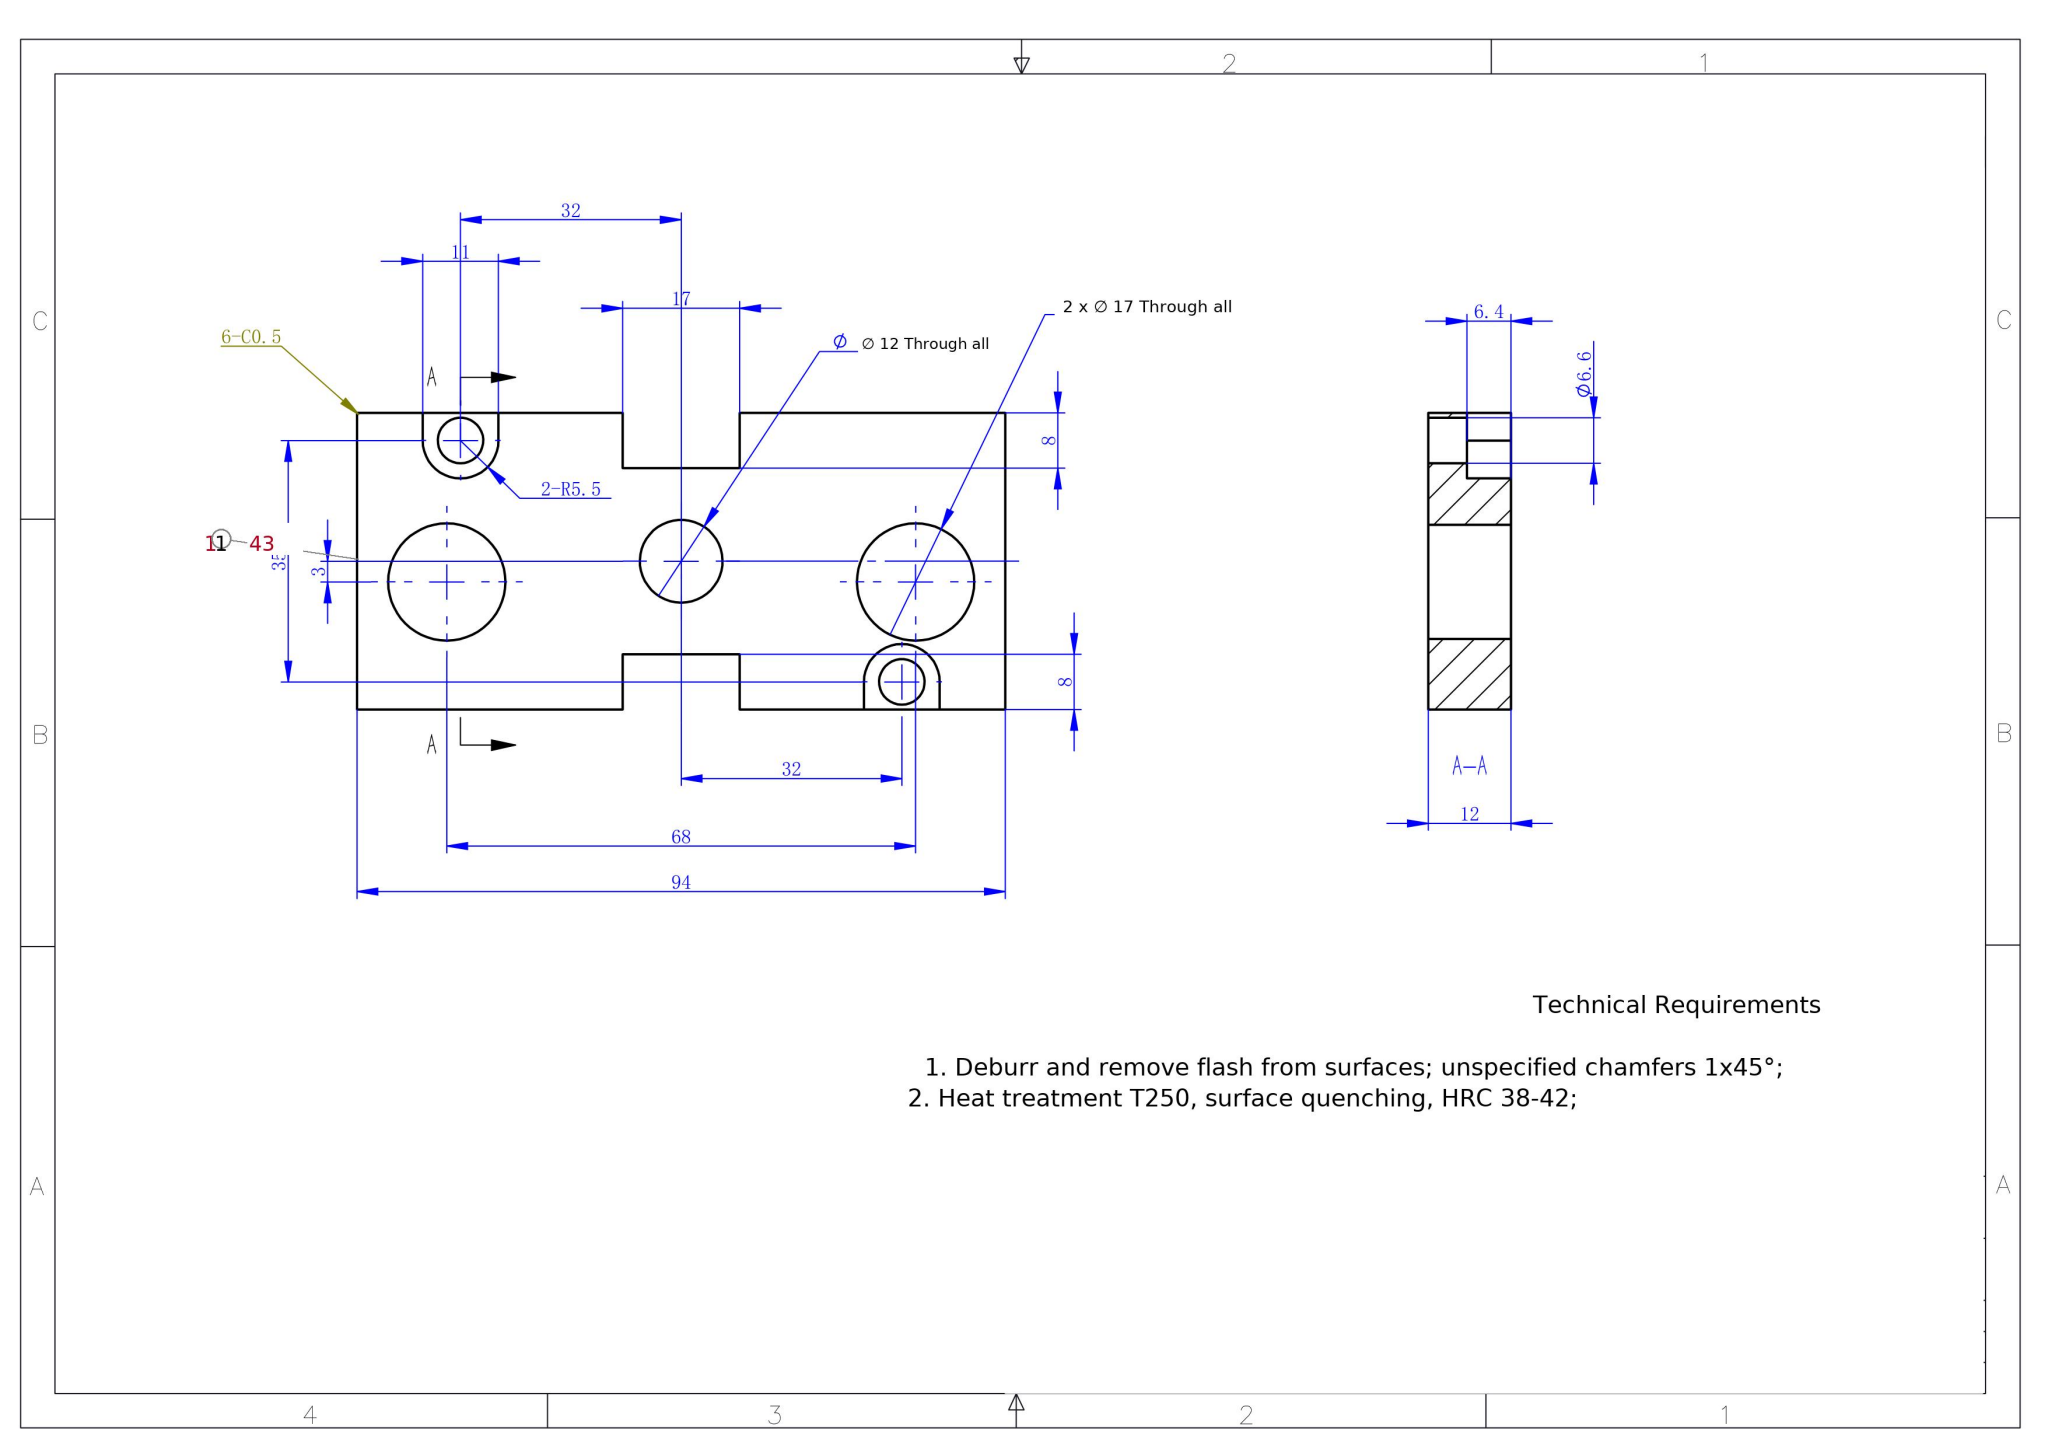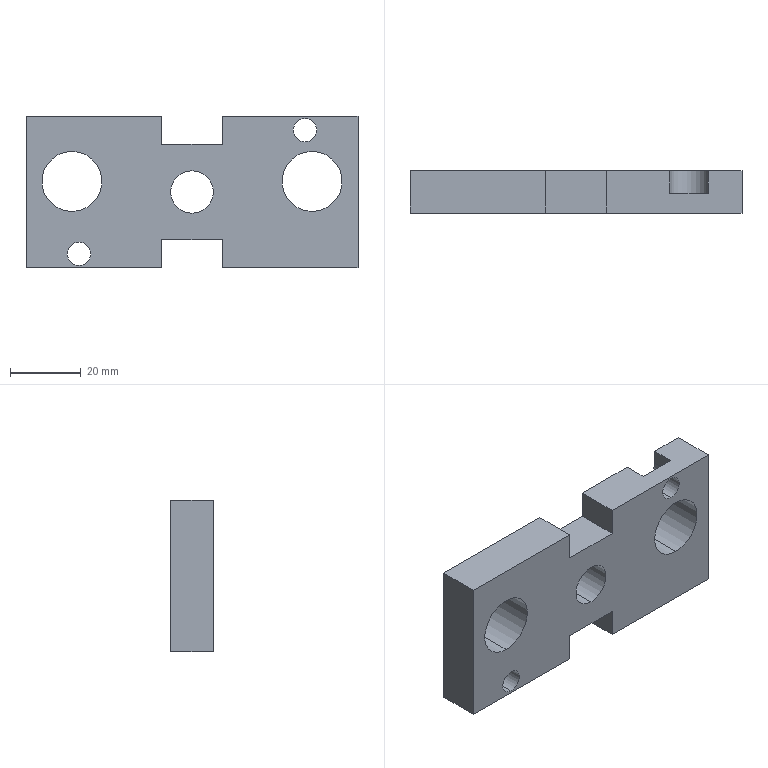Part | SolidWorks | mm | 1 solid | 33 faces | box 94 x 12 x 43 mm | volume 36881 mm3 | plane 20 | cylinder 13 | commonest cylinder face diameters 6.6 x4 17 x4 11 x3 12 x2
build123d program:
from build123d import *

# Parameters (mm, degrees)
SKETCH1_W                                       = 94
SKETCH1_H                                       = 43
BOSS_EXTRUDE1_DEPTH                             = 12
F_6_0_6_DIAMETER_HOLE1_D                        = 17
F_6_0_6_DIAMETER_HOLE2_D                        = 12
M6_HEX_SOCKET_HEAD_CAP_SCREW_CBORE1_D           = 6.6
M6_HEX_SOCKET_HEAD_CAP_SCREW_CBORE1_CBORE_D     = 11
M6_HEX_SOCKET_HEAD_CAP_SCREW_CBORE1_CBORE_DEPTH = 6.4
CUT_EXTRUDE2_DEPTH                              = 6.4
SKETCH10_W                                      = 17
SKETCH10_H                                      = 8
CUT_EXTRUDE3_DEPTH                              = 54.059


with BuildPart() as part:
    # Sketch1 → Boss-Extrude1 (new body)
    with BuildSketch(Plane(origin=(0, 0, 0), x_dir=(1, 0, 0), z_dir=(0, 1, 0))):
        Rectangle(SKETCH1_W, SKETCH1_H)
    extrude(amount=BOSS_EXTRUDE1_DEPTH)

    # 6.0 _6_ Diameter Hole1 (through all)
    with Locations(Plane(origin=(0, 12, 0), x_dir=(1, 0, 0), z_dir=(0, 1, 0))):
        with Locations((-34, -3), (34, -3)):
            Hole(F_6_0_6_DIAMETER_HOLE1_D / 2)

    # 6.0 _6_ Diameter Hole2 (through all)
    with Locations(Plane(origin=(0, 12, 0), x_dir=(1, 0, 0), z_dir=(0, 1, 0))):
        with Locations((0, 0)):
            Hole(F_6_0_6_DIAMETER_HOLE2_D / 2)

    # M6 Hex Socket Head Cap Screw CBORE1 (through all)
    with Locations(Plane(origin=(0, 12, 0), x_dir=(1, 0, 0), z_dir=(0, 1, 0))):
        with Locations((-32, 17.5), (32, -17.5)):
            CounterBoreHole(M6_HEX_SOCKET_HEAD_CAP_SCREW_CBORE1_D / 2, M6_HEX_SOCKET_HEAD_CAP_SCREW_CBORE1_CBORE_D / 2, M6_HEX_SOCKET_HEAD_CAP_SCREW_CBORE1_CBORE_DEPTH)

    # Sketch9 → Cut-Extrude2 (cut)
    with BuildSketch(Plane(origin=(0, 12, 0), x_dir=(1, 0, 0), z_dir=(0, 1, 0))):
        with BuildLine():
            Line((-37.5, 17.5), (-37.5, 30.416))
            ThreePointArc((-37.5, 30.416), (-32, 35.916), (-26.5, 30.416))
            Line((-26.5, 30.416), (-26.5, 17.5))
            ThreePointArc((-26.5, 17.5), (-32, 12), (-37.5, 17.5))
        make_face()
        with BuildLine():
            Line((37.5, -17.5), (37.5, -32.022))
            ThreePointArc((37.5, -32.022), (32, -37.522), (26.5, -32.022))
            Line((26.5, -32.022), (26.5, -17.5))
            ThreePointArc((26.5, -17.5), (32, -12), (37.5, -17.5))
        make_face()
    extrude(amount=-CUT_EXTRUDE2_DEPTH, mode=Mode.SUBTRACT)

    # Sketch10 → Cut-Extrude3 (cut, through all)
    with BuildSketch(Plane.XZ):
        with Locations((0, 17.5)):
            Rectangle(SKETCH10_W, SKETCH10_H)
        with Locations((0, -17.5)):
            Rectangle(SKETCH10_W, SKETCH10_H)
    extrude(amount=-CUT_EXTRUDE3_DEPTH, mode=Mode.SUBTRACT)


solid = part.part